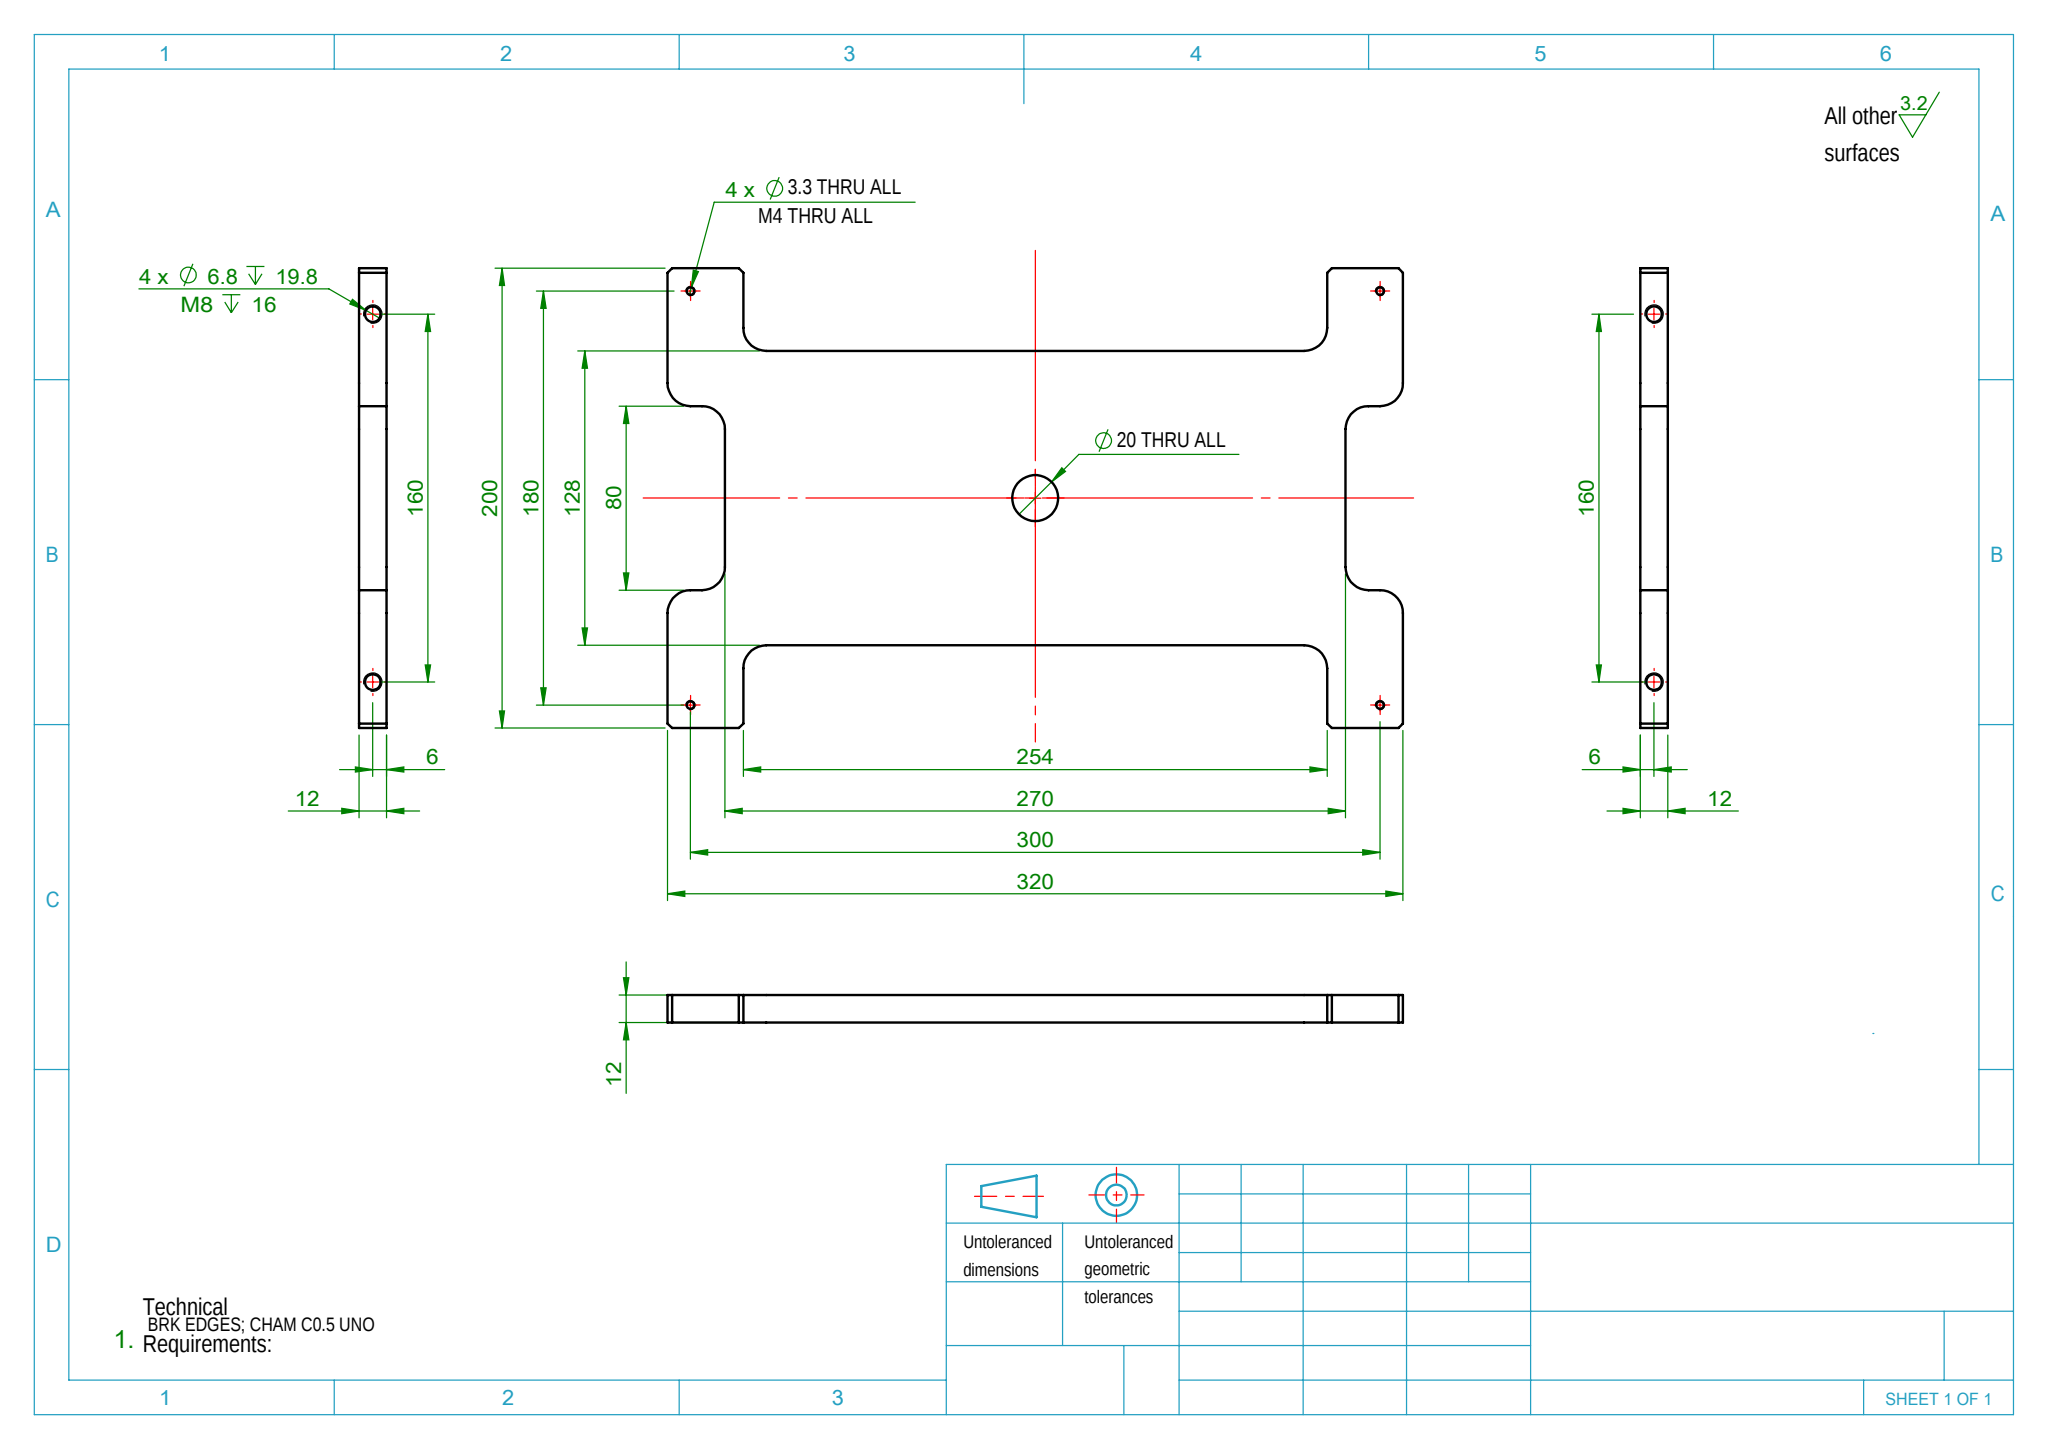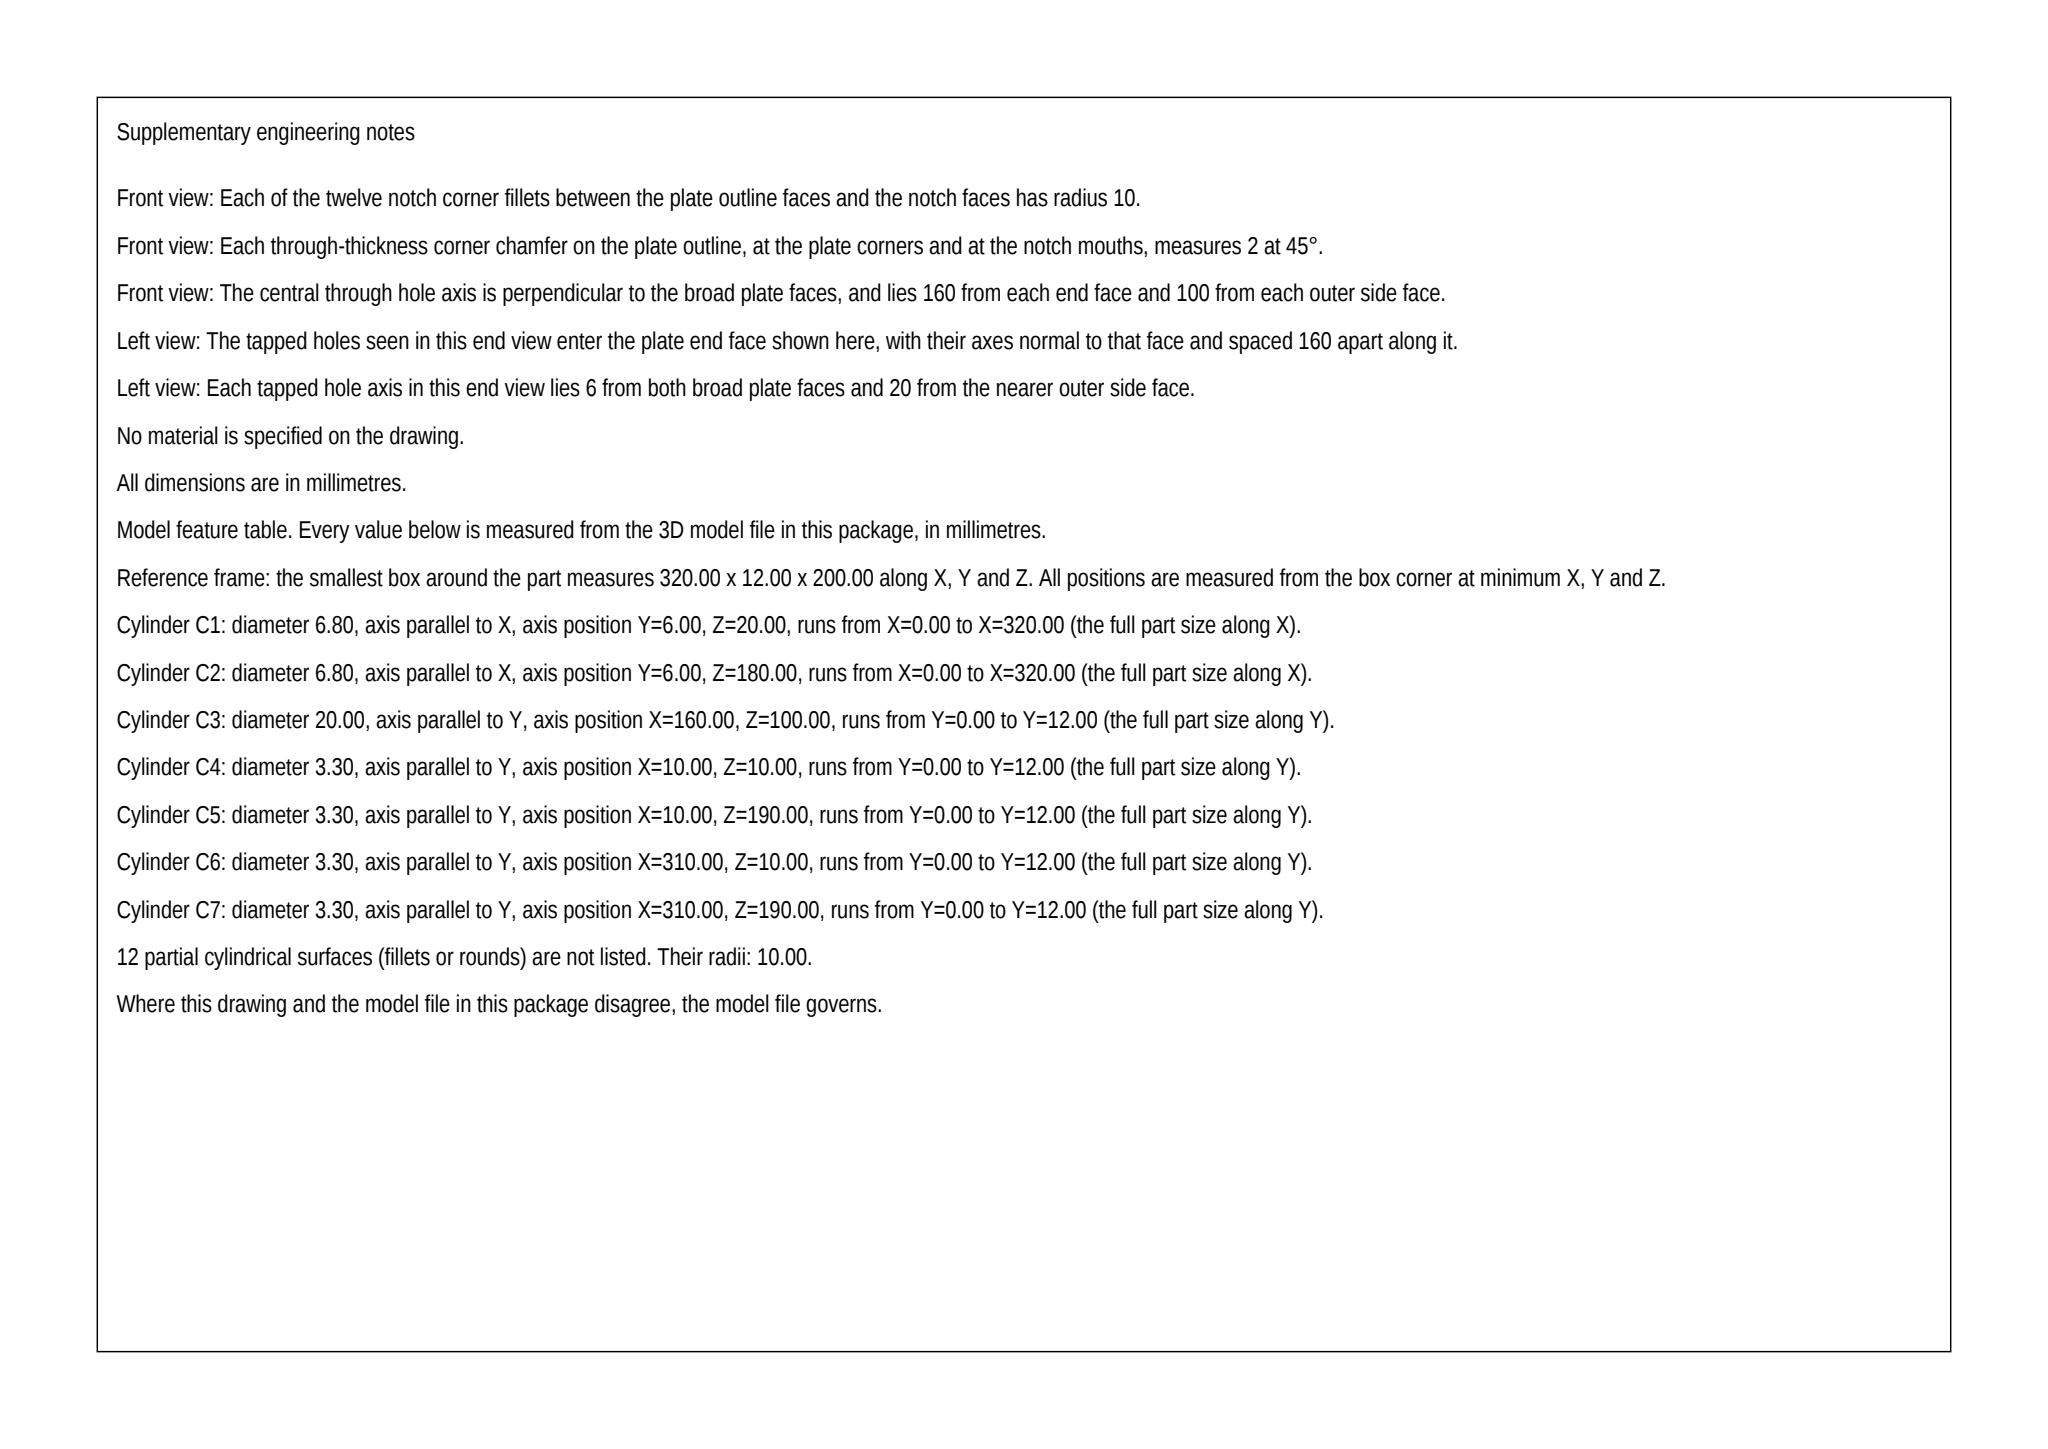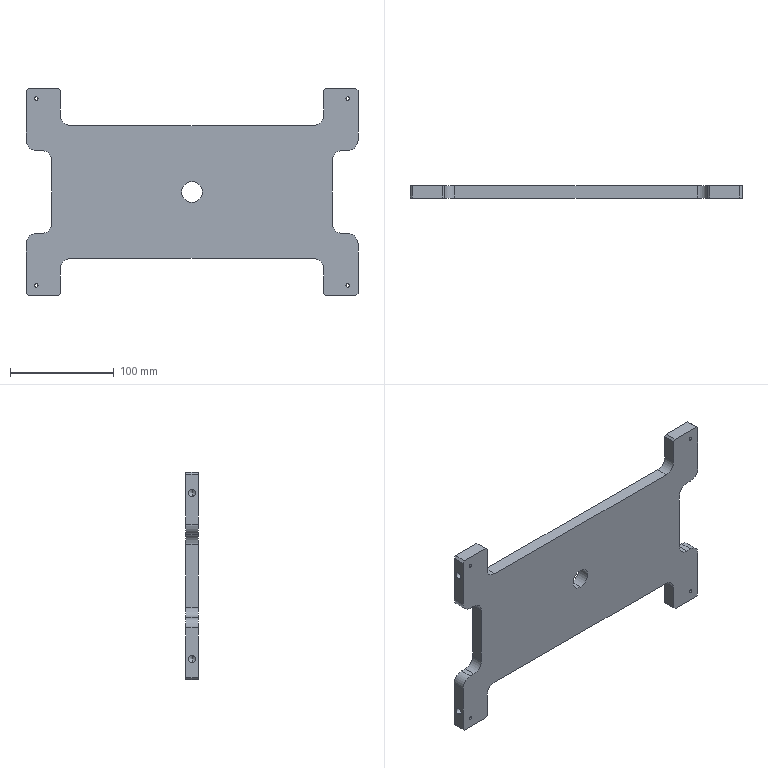Part | SolidWorks | mm | 1 solid | 68 faces | box 320 x 12 x 200 mm | volume 494234 mm3 | cylinder 30 | plane 30 | cone 8 | commonest cylinder face diameters 20 x14 3.3 x8 6.8 x8
build123d program:
from build123d import *

# Parameters (mm, degrees)
SKETCH1_W                  = 320
SKETCH1_H                  = 200
BOSS_EXTRUDE1_DEPTH        = 12
SKETCH2_W                  = 254
SKETCH2_H                  = 36
SKETCH2_W_2                = 25
SKETCH2_H_2                = 80
CUT_EXTRUDE1_DEPTH         = 190.061
FILLET1_R                  = 10
M8_TAPPED_HOLE1_AT_2_COUNT = 2
M8_TAPPED_HOLE1_AT_2_PITCH = 160
F_20_0_20_DIAMETER_HOLE1_D = 20
M4_TAPPED_HOLE1_D          = 3.3
CHAMFER1_SIZE              = 2


with BuildPart() as part:
    # Sketch1 → Boss-Extrude1 (new body)
    with BuildSketch(Plane(origin=(0, 0, 0), x_dir=(1, 0, 0), z_dir=(0, 1, 0))):
        Rectangle(SKETCH1_W, SKETCH1_H)
    extrude(amount=BOSS_EXTRUDE1_DEPTH)

    # Sketch2 → Cut-Extrude1 (cut, through all)
    with BuildSketch(Plane(origin=(0, 12, 0), x_dir=(1, 0, 0), z_dir=(0, 1, 0))):
        with Locations((0, 82)):
            Rectangle(SKETCH2_W, SKETCH2_H)
        with Locations((0, -82)):
            Rectangle(SKETCH2_W, SKETCH2_H)
        with Locations((-147.5, 0)):
            Rectangle(SKETCH2_W_2, SKETCH2_H_2)
        with Locations((147.5, 0)):
            Rectangle(SKETCH2_W_2, SKETCH2_H_2)
    extrude(amount=-CUT_EXTRUDE1_DEPTH, mode=Mode.SUBTRACT)

    # Fillet1
    fillet1_edges = [part.edges().sort_by_distance(p)[0] for p in [
        (127, 6, -64),
        (-127, 6, -64),
        (127, 6, 64),
        (-127, 6, 64),
        (-160, 6, 40),
        (-160, 6, -40),
        (-135, 6, -40),
        (-135, 6, 40),
        (160, 6, -40),
        (160, 6, 40),
        (135, 6, 40),
        (135, 6, -40),
    ]]
    fillet(fillet1_edges, radius=FILLET1_R)

    # Sketch4 → M8 Tapped Hole1 (revolve, cut)
    with BuildSketch(Plane(origin=(160, 6, 80), x_dir=(0, 0, -1), z_dir=(0, 1, 0))):
        Polygon((0, 0), (0, 21.793), (3.4, 19.75), (3.4, 0), align=None)
    m8_tapped_hole1 = revolve(axis=Axis((166.35, 6, 80), (-1, 0, 0)), mode=Mode.SUBTRACT)

    # M8 Tapped Hole1 at 2: M8 Tapped Hole1 ×2
    with Locations(*[(0, 0, -i * M8_TAPPED_HOLE1_AT_2_PITCH) for i in range(1, M8_TAPPED_HOLE1_AT_2_COUNT)]):
        add(m8_tapped_hole1, mode=Mode.SUBTRACT)

    # Mirror1: M8 Tapped Hole1 across plane
    add(m8_tapped_hole1.mirror(Plane(origin=(0, 0, 0), x_dir=(0, 0, 1), z_dir=(1, 0, 0))), mode=Mode.SUBTRACT)

    # Mirror1 copy 1 sketch → Mirror1 copy 1 (revolve, cut)
    with BuildSketch(Plane(origin=(-160, 6, -80), x_dir=(0, 0, -1), z_dir=(0, 1, 0))):
        Polygon((0, 0), (0, -21.793), (3.4, -19.75), (3.4, 0), align=None)
    revolve(axis=Axis((-166.35, 6, -80), (-1, 0, 0)), mode=Mode.SUBTRACT)

    # 20.0 _20_ Diameter Hole1 (through all)
    with Locations(Plane(origin=(0, 12, 0), x_dir=(1, 0, 0), z_dir=(0, 1, 0))):
        with Locations((0, 0)):
            Hole(F_20_0_20_DIAMETER_HOLE1_D / 2)

    # M4 Tapped Hole1 (through all)
    with Locations(Plane(origin=(0, 12, 0), x_dir=(1, 0, 0), z_dir=(0, 1, 0))):
        with Locations((-150, 90), (-150, -90), (150, -90), (150, 90)):
            Hole(M4_TAPPED_HOLE1_D / 2)

    # Chamfer1
    chamfer1_edges = [part.edges().sort_by_distance(p)[0] for p in [
        (127, 6, -100),
        (-127, 6, -100),
        (127, 6, 100),
        (-127, 6, 100),
        (160, 6, 100),
        (-160, 6, 100),
        (-160, 6, -100),
        (160, 6, -100),
    ]]
    chamfer(chamfer1_edges, length=CHAMFER1_SIZE)


solid = part.part